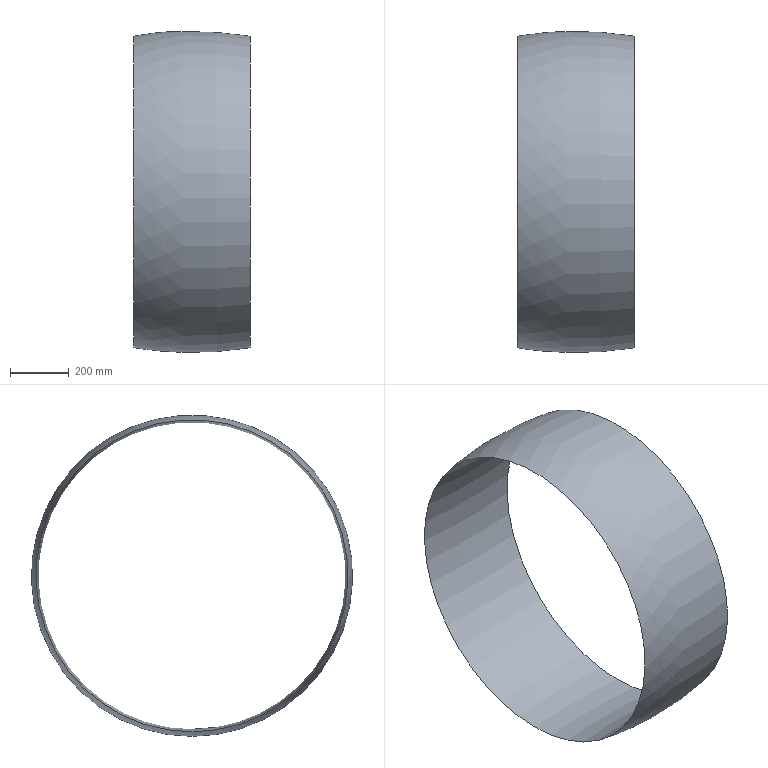Component | NX | MAIN_HOUSING | 1 solid | 2 faces | box 396.46 x 1092.34 x 1092.34 mm | volume 22799491 mm3 | other 2
STEP:
#1=CARTESIAN_POINT('',(0.,0.,0.));
#2=DIRECTION('',(0.,0.,1.));
#3=DIRECTION('',(1.,0.,0.));
#4=AXIS2_PLACEMENT_3D('',#1,#2,#3);
#5=CARTESIAN_POINT('',(5.293,0.,-530.));
#6=VERTEX_POINT('',#5);
#7=CARTESIAN_POINT('',(5.293,0.,-0.));
#8=DIRECTION('',(1.,0.,0.));
#9=DIRECTION('',(0.,0.,-1.));
#10=AXIS2_PLACEMENT_3D('',#7,#8,#9);
#11=CIRCLE('',#10,530.);
#12=CARTESIAN_POINT('',(401.751,0.,530.));
#13=CARTESIAN_POINT('',(201.751,0.,562.339));
#14=CARTESIAN_POINT('',(5.293,0.,530.));
#15=B_SPLINE_CURVE_WITH_KNOTS('',2,(#12,#13,#14),.UNSPECIFIED.,.F.,.F.,(3,3),(0.,1.),.PIECEWISE_BEZIER_KNOTS.);
#16=CARTESIAN_POINT('',(386.987,0.,-0.));
#17=DIRECTION('',(1.,0.,0.));
#18=AXIS1_PLACEMENT('',#16,#17);
#19=SURFACE_OF_REVOLUTION('',#15,#18);
#20=CARTESIAN_POINT('',(3.142,1.));
#21=DIRECTION('',(1.,0.));
#22=VECTOR('',#21,1.);
#23=LINE('',#20,#22);
#24=(GEOMETRIC_REPRESENTATION_CONTEXT(2)PARAMETRIC_REPRESENTATION_CONTEXT()REPRESENTATION_CONTEXT('',''));
#25=DEFINITIONAL_REPRESENTATION('',(#23),#24);
#26=PCURVE('',#19,#25);
#27=CARTESIAN_POINT('',(5.293,0.,530.));
#28=CARTESIAN_POINT('',(205.293,0.,510.786));
#29=CARTESIAN_POINT('',(401.751,0.,530.));
#30=B_SPLINE_CURVE_WITH_KNOTS('',2,(#27,#28,#29),.UNSPECIFIED.,.F.,.F.,(3,3),(0.,1.),.PIECEWISE_BEZIER_KNOTS.);
#31=CARTESIAN_POINT('',(386.987,0.,-0.));
#32=DIRECTION('',(1.,0.,0.));
#33=AXIS1_PLACEMENT('',#31,#32);
#34=SURFACE_OF_REVOLUTION('',#30,#33);
#35=CARTESIAN_POINT('',(3.142,0.));
#36=DIRECTION('',(1.,0.));
#37=VECTOR('',#36,1.);
#38=LINE('',#35,#37);
#39=(GEOMETRIC_REPRESENTATION_CONTEXT(2)PARAMETRIC_REPRESENTATION_CONTEXT()REPRESENTATION_CONTEXT('',''));
#40=DEFINITIONAL_REPRESENTATION('',(#38),#39);
#41=PCURVE('',#34,#40);
#42=SURFACE_CURVE('',#11,(#26,#41),.PCURVE_S1.);
#43=EDGE_CURVE('',#6,#6,#42,.T.);
#44=ORIENTED_EDGE('',*,*,#43,.F.);
#45=CARTESIAN_POINT('',(401.751,0.,-530.));
#46=VERTEX_POINT('',#45);
#47=CARTESIAN_POINT('',(401.751,-0.,-530.));
#48=CARTESIAN_POINT('',(201.751,-0.,-562.339));
#49=CARTESIAN_POINT('',(5.293,-0.,-530.));
#50=B_SPLINE_CURVE_WITH_KNOTS('',2,(#47,#48,#49),.UNSPECIFIED.,.F.,.F.,(3,3),(-0.,1.),.PIECEWISE_BEZIER_KNOTS.);
#51=CARTESIAN_POINT('',(3.142,0.));
#52=DIRECTION('',(0.,1.));
#53=VECTOR('',#52,1.);
#54=LINE('',#51,#53);
#55=(GEOMETRIC_REPRESENTATION_CONTEXT(2)PARAMETRIC_REPRESENTATION_CONTEXT()REPRESENTATION_CONTEXT('',''));
#56=DEFINITIONAL_REPRESENTATION('',(#54),#55);
#57=PCURVE('',#19,#56);
#58=CARTESIAN_POINT('',(9.425,0.));
#59=DIRECTION('',(0.,1.));
#60=VECTOR('',#59,1.);
#61=LINE('',#58,#60);
#62=(GEOMETRIC_REPRESENTATION_CONTEXT(2)PARAMETRIC_REPRESENTATION_CONTEXT()REPRESENTATION_CONTEXT('',''));
#63=DEFINITIONAL_REPRESENTATION('',(#61),#62);
#64=PCURVE('',#19,#63);
#65=SEAM_CURVE('',#50,(#57,#64),.PCURVE_S1.);
#66=EDGE_CURVE('',#46,#6,#65,.T.);
#67=ORIENTED_EDGE('',*,*,#66,.F.);
#68=CARTESIAN_POINT('',(401.751,0.,-0.));
#69=DIRECTION('',(-1.,0.,0.));
#70=DIRECTION('',(0.,0.,-1.));
#71=AXIS2_PLACEMENT_3D('',#68,#69,#70);
#72=CIRCLE('',#71,530.);
#73=CARTESIAN_POINT('',(9.425,-0.));
#74=DIRECTION('',(-1.,0.));
#75=VECTOR('',#74,1.);
#76=LINE('',#73,#75);
#77=(GEOMETRIC_REPRESENTATION_CONTEXT(2)PARAMETRIC_REPRESENTATION_CONTEXT()REPRESENTATION_CONTEXT('',''));
#78=DEFINITIONAL_REPRESENTATION('',(#76),#77);
#79=PCURVE('',#19,#78);
#80=CARTESIAN_POINT('',(9.425,1.));
#81=DIRECTION('',(-1.,0.));
#82=VECTOR('',#81,1.);
#83=LINE('',#80,#82);
#84=(GEOMETRIC_REPRESENTATION_CONTEXT(2)PARAMETRIC_REPRESENTATION_CONTEXT()REPRESENTATION_CONTEXT('',''));
#85=DEFINITIONAL_REPRESENTATION('',(#83),#84);
#86=PCURVE('',#34,#85);
#87=SURFACE_CURVE('',#72,(#79,#86),.PCURVE_S1.);
#88=EDGE_CURVE('',#46,#46,#87,.T.);
#89=ORIENTED_EDGE('',*,*,#88,.F.);
#90=ORIENTED_EDGE('',*,*,#66,.T.);
#91=EDGE_LOOP('',(#44,#67,#89,#90));
#92=FACE_BOUND('',#91,.F.);
#93=ADVANCED_FACE('',(#92),#19,.F.);
#94=ORIENTED_EDGE('',*,*,#88,.T.);
#95=CARTESIAN_POINT('',(5.293,-0.,-530.));
#96=CARTESIAN_POINT('',(205.293,-0.,-510.786));
#97=CARTESIAN_POINT('',(401.751,-0.,-530.));
#98=B_SPLINE_CURVE_WITH_KNOTS('',2,(#95,#96,#97),.UNSPECIFIED.,.F.,.F.,(3,3),(0.,1.),.PIECEWISE_BEZIER_KNOTS.);
#99=CARTESIAN_POINT('',(3.142,0.));
#100=DIRECTION('',(0.,1.));
#101=VECTOR('',#100,1.);
#102=LINE('',#99,#101);
#103=(GEOMETRIC_REPRESENTATION_CONTEXT(2)PARAMETRIC_REPRESENTATION_CONTEXT()REPRESENTATION_CONTEXT('',''));
#104=DEFINITIONAL_REPRESENTATION('',(#102),#103);
#105=PCURVE('',#34,#104);
#106=CARTESIAN_POINT('',(9.425,0.));
#107=DIRECTION('',(0.,1.));
#108=VECTOR('',#107,1.);
#109=LINE('',#106,#108);
#110=(GEOMETRIC_REPRESENTATION_CONTEXT(2)PARAMETRIC_REPRESENTATION_CONTEXT()REPRESENTATION_CONTEXT('',''));
#111=DEFINITIONAL_REPRESENTATION('',(#109),#110);
#112=PCURVE('',#34,#111);
#113=SEAM_CURVE('',#98,(#105,#112),.PCURVE_S1.);
#114=EDGE_CURVE('',#6,#46,#113,.T.);
#115=ORIENTED_EDGE('',*,*,#114,.F.);
#116=ORIENTED_EDGE('',*,*,#43,.T.);
#117=ORIENTED_EDGE('',*,*,#114,.T.);
#118=EDGE_LOOP('',(#94,#115,#116,#117));
#119=FACE_BOUND('',#118,.F.);
#120=ADVANCED_FACE('',(#119),#34,.F.);
#121=CLOSED_SHELL('',(#93,#120));
#122=MANIFOLD_SOLID_BREP('',#121);
#123=(LENGTH_UNIT()NAMED_UNIT(*)SI_UNIT(.MILLI.,.METRE.));
#124=UNCERTAINTY_MEASURE_WITH_UNIT(LENGTH_MEASURE(0.00001),#123,'','');
#125=(NAMED_UNIT(*)PLANE_ANGLE_UNIT()SI_UNIT($,.RADIAN.));
#126=(NAMED_UNIT(*)SI_UNIT($,.STERADIAN.)SOLID_ANGLE_UNIT());
#127=(GEOMETRIC_REPRESENTATION_CONTEXT(3)GLOBAL_UNCERTAINTY_ASSIGNED_CONTEXT((#124))GLOBAL_UNIT_ASSIGNED_CONTEXT((#123,#125,#126))REPRESENTATION_CONTEXT('',''));
#128=ADVANCED_BREP_SHAPE_REPRESENTATION('',(#4,#122),#127);